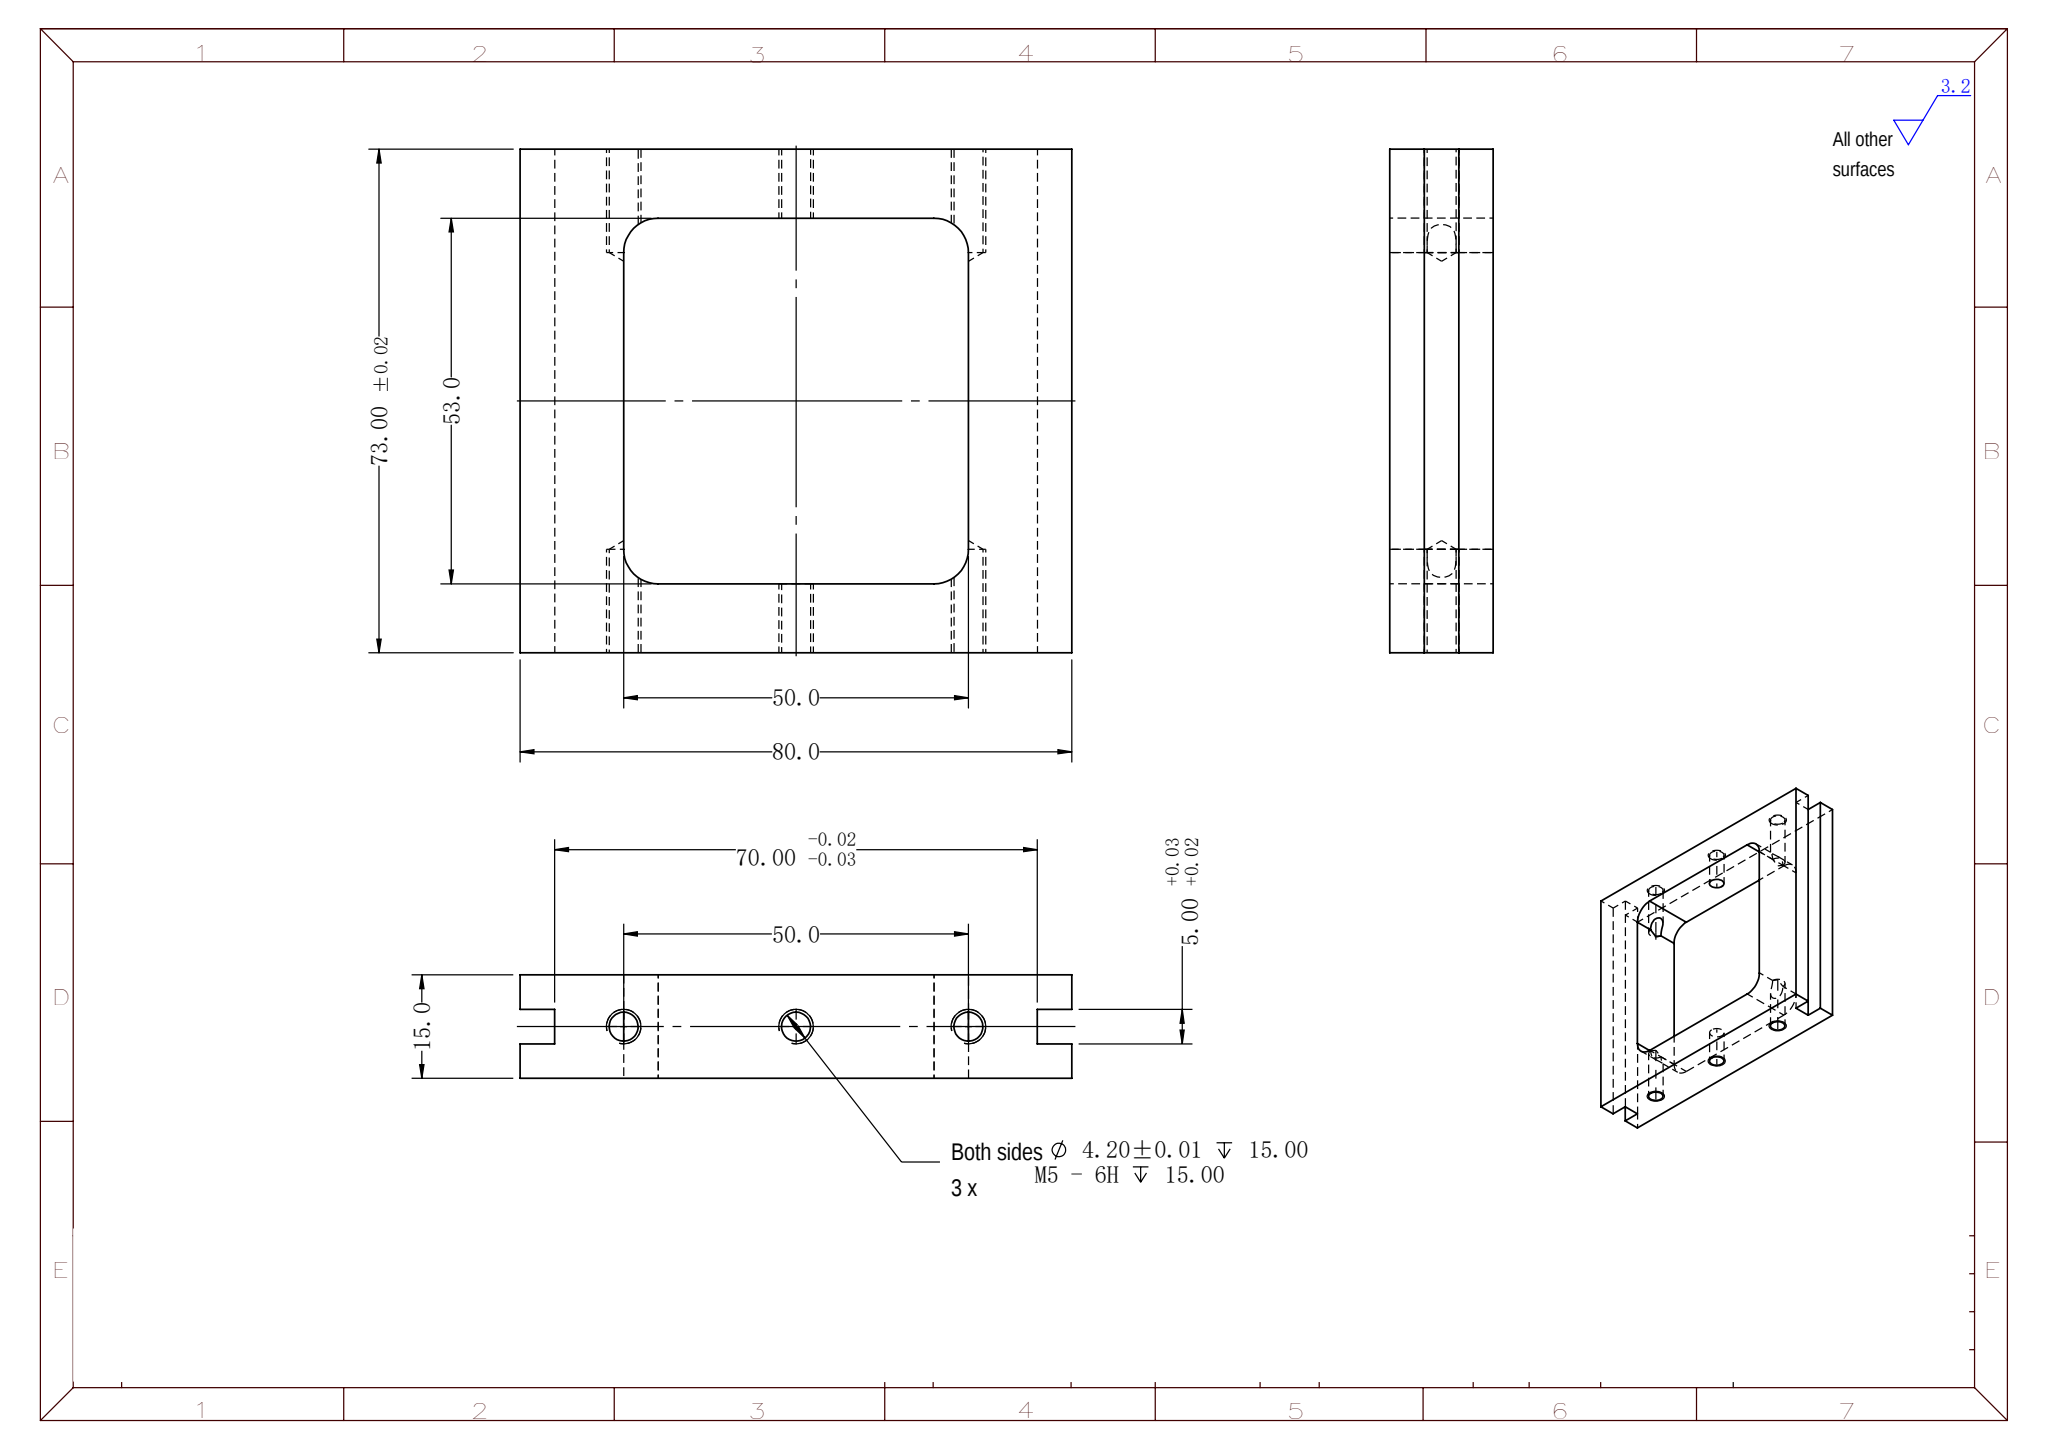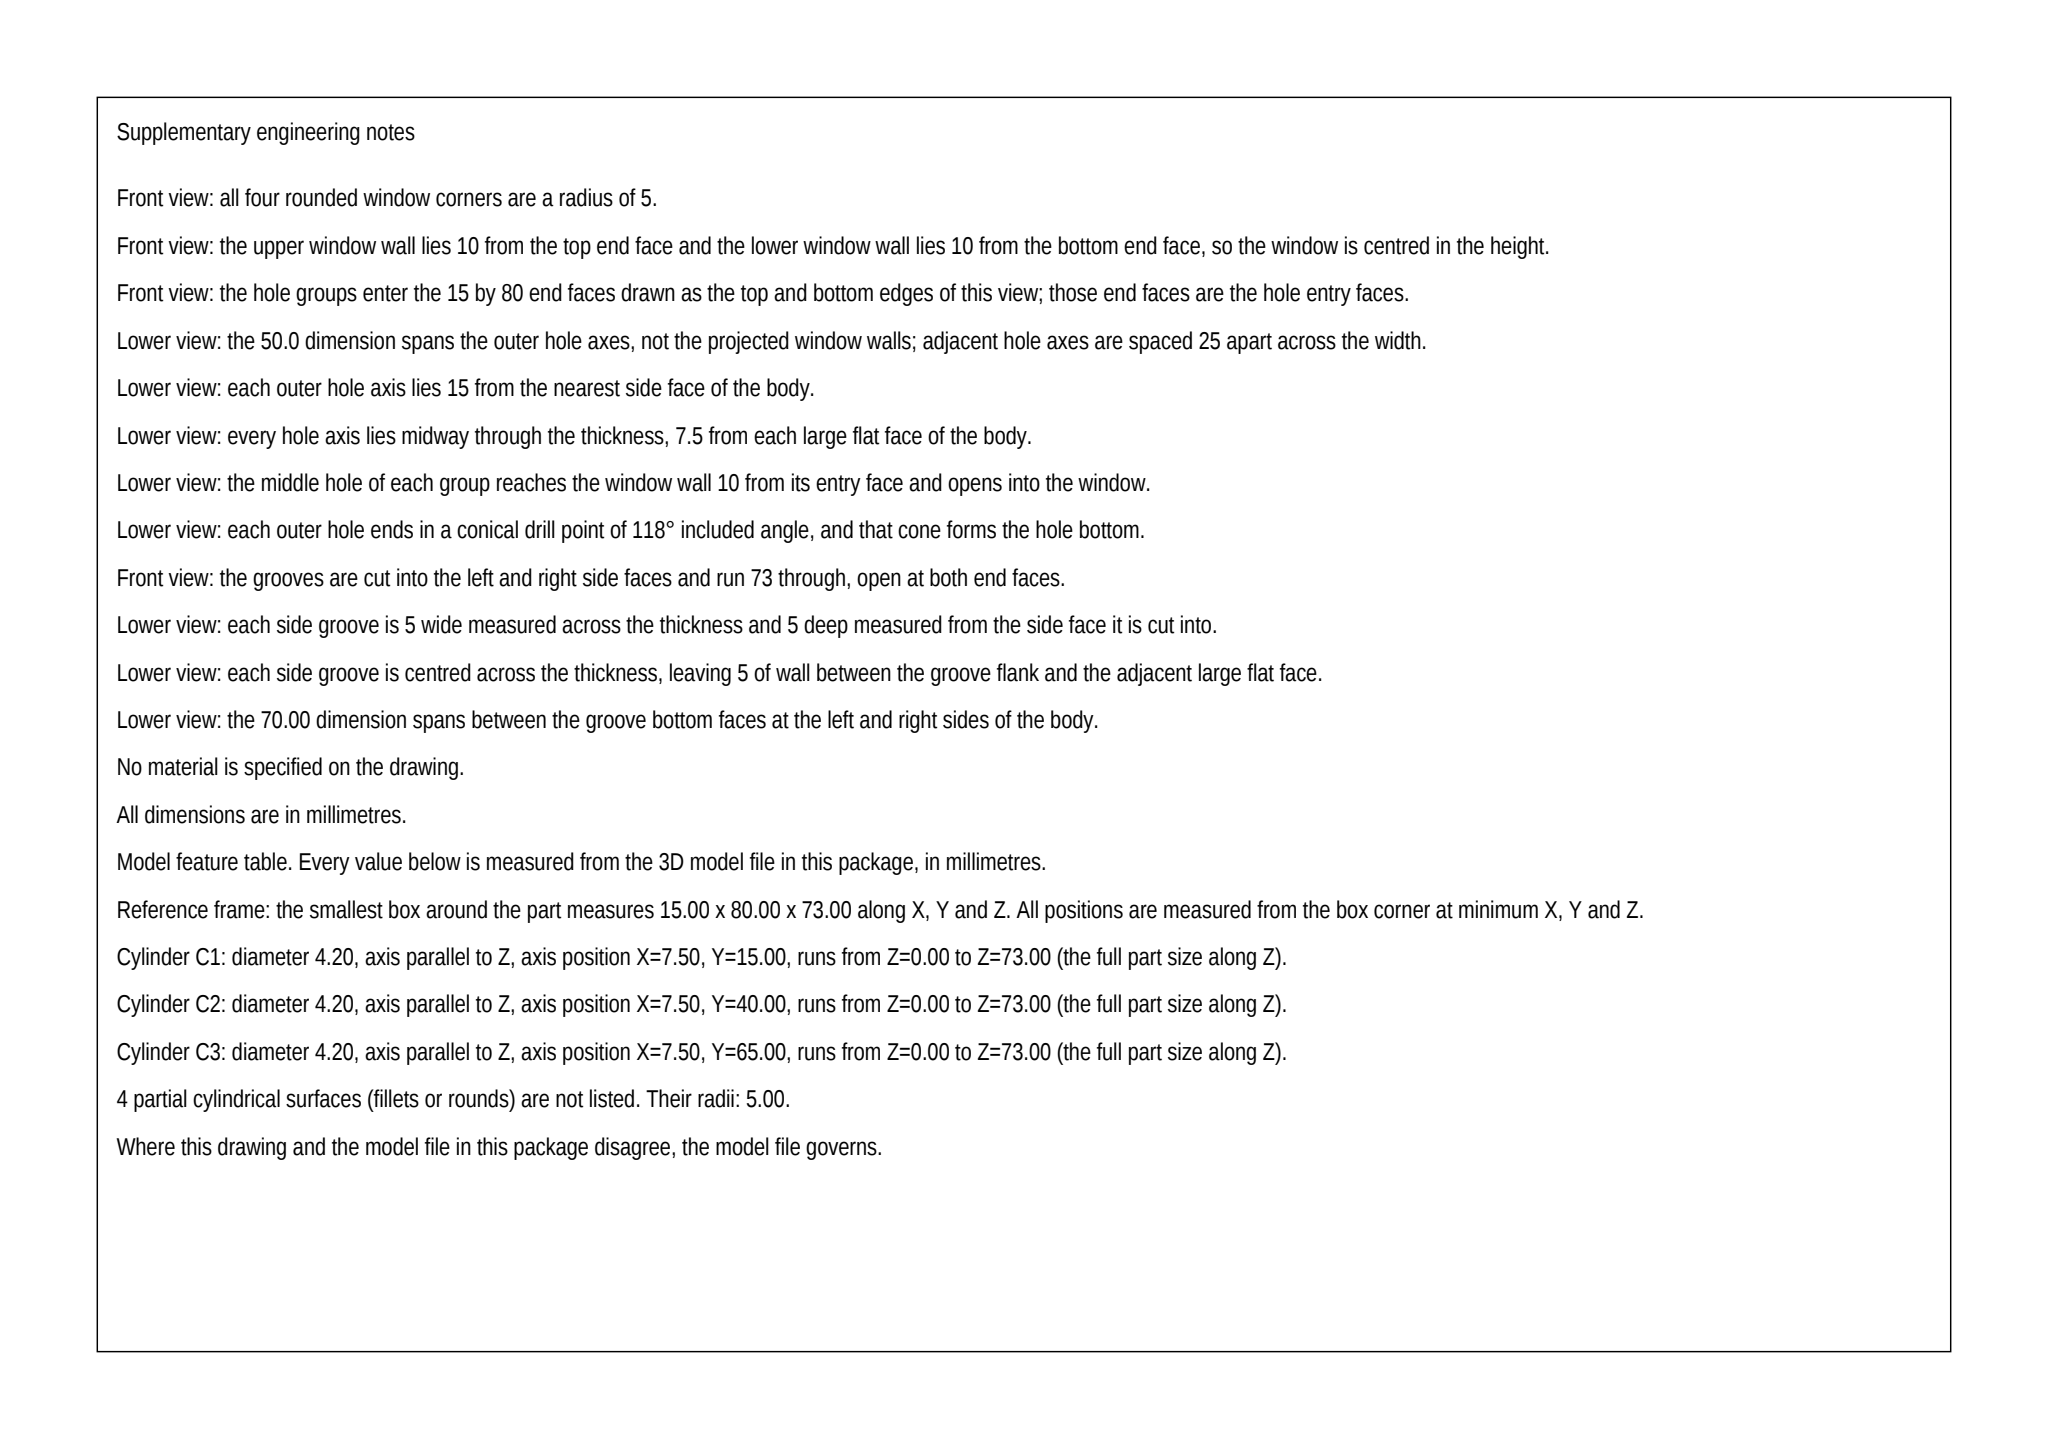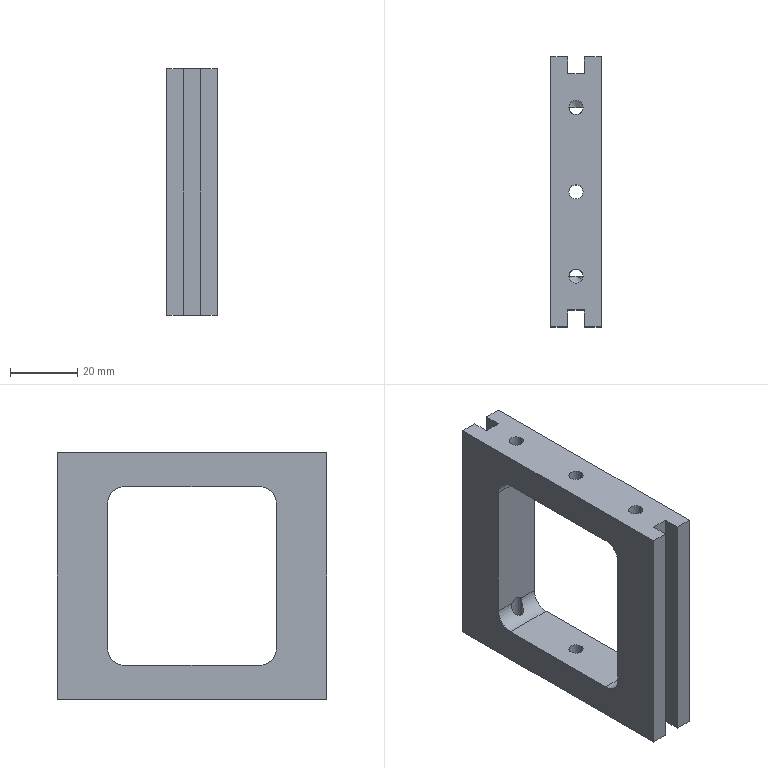Part | SolidWorks | mm | 1 solid | 38 faces | box 15 x 80 x 73 mm | volume 43475 mm3 | plane 18 | cylinder 16 | cone 4 | commonest cylinder face diameters 4.2 x12 10 x4
Drawing notes:
CENTRE M5 THD DP 10 BOTH SIDES (OUTER 2 HOLES DP 15) | from the solid: Ø4.2 z-axis holes at x=7.5: y=15 & y=65 length 15, y=40 length 10
50.0 x 53.0 R5 POCKET THRU 15 THK | from the solid: Pocket faces y=15/65 (50 wide), z=10/63 (53 high); plate x=0 to 15 thk, no pocket floor plane
build123d program:
from build123d import *

# Parameters (mm, degrees)
SKETCH1_W             = 15
SKETCH1_H             = 80
BOSS_EXTRUDE1_DEPTH   = 36.5
SKETCH9_W             = 53
SKETCH9_H             = 50
CUT_EXTRUDE1_DEPTH    = 57.189
SKETCH10_W            = 5
SKETCH10_H            = 5
CUT_EXTRUDE2_DEPTH    = 84.578
FILLET1_R             = 5
M5_TAPPED_HOLE1_D     = 4.2
M5_TAPPED_HOLE1_DEPTH = 15
M5_TAPPED_HOLE1_TIP   = 1.262
M5_TAPPED_HOLE2_D     = 4.2
M5_TAPPED_HOLE2_DEPTH = 15
M5_TAPPED_HOLE2_TIP   = 1.262


with BuildPart() as part:
    # Sketch1 → Boss-Extrude1 (new, symmetric)
    with BuildSketch(Plane.XY):
        Rectangle(SKETCH1_W, SKETCH1_H)
    extrude(amount=BOSS_EXTRUDE1_DEPTH, both=True)

    # Sketch9 → Cut-Extrude1 (cut, through all)
    with BuildSketch(Plane(origin=(7.5, 0, 0), x_dir=(0, 0, -1), z_dir=(1, 0, 0))):
        Rectangle(SKETCH9_W, SKETCH9_H)
    extrude(amount=-CUT_EXTRUDE1_DEPTH, mode=Mode.SUBTRACT)

    # Sketch10 → Cut-Extrude2 (cut, through all)
    with BuildSketch(Plane.XY.offset(36.5)):
        with Locations((0, 37.5)):
            Rectangle(SKETCH10_W, SKETCH10_H)
        with Locations((0, -37.5)):
            Rectangle(SKETCH10_W, SKETCH10_H)
    extrude(amount=-CUT_EXTRUDE2_DEPTH, mode=Mode.SUBTRACT)

    # Fillet1
    fillet1_edges = [part.edges().sort_by_distance(p)[0] for p in [
        (0, 25, -26.5),
        (0, -25, -26.5),
        (0, -25, 26.5),
        (0, 25, 26.5),
    ]]
    fillet(fillet1_edges, radius=FILLET1_R)

    # M5 Tapped Hole1
    with Locations(Plane.XY.offset(36.5)):
        with Locations((0, -25), (0, 0), (0, 25)):
            Hole(M5_TAPPED_HOLE1_D / 2, depth=M5_TAPPED_HOLE1_DEPTH)
            with Locations((0, 0, -(M5_TAPPED_HOLE1_DEPTH + M5_TAPPED_HOLE1_TIP / 2))):  # 118° drill point
                Cone(0, M5_TAPPED_HOLE1_D / 2, M5_TAPPED_HOLE1_TIP, mode=Mode.SUBTRACT)

    # M5 Tapped Hole2
    with Locations(Plane(origin=(0, 0, -36.5), x_dir=(-1, 0, 0), z_dir=(0, 0, -1))):
        with Locations((0, -25), (0, 0), (0, 25)):
            Hole(M5_TAPPED_HOLE2_D / 2, depth=M5_TAPPED_HOLE2_DEPTH)
            with Locations((0, 0, -(M5_TAPPED_HOLE2_DEPTH + M5_TAPPED_HOLE2_TIP / 2))):  # 118° drill point
                Cone(0, M5_TAPPED_HOLE2_D / 2, M5_TAPPED_HOLE2_TIP, mode=Mode.SUBTRACT)


solid = part.part